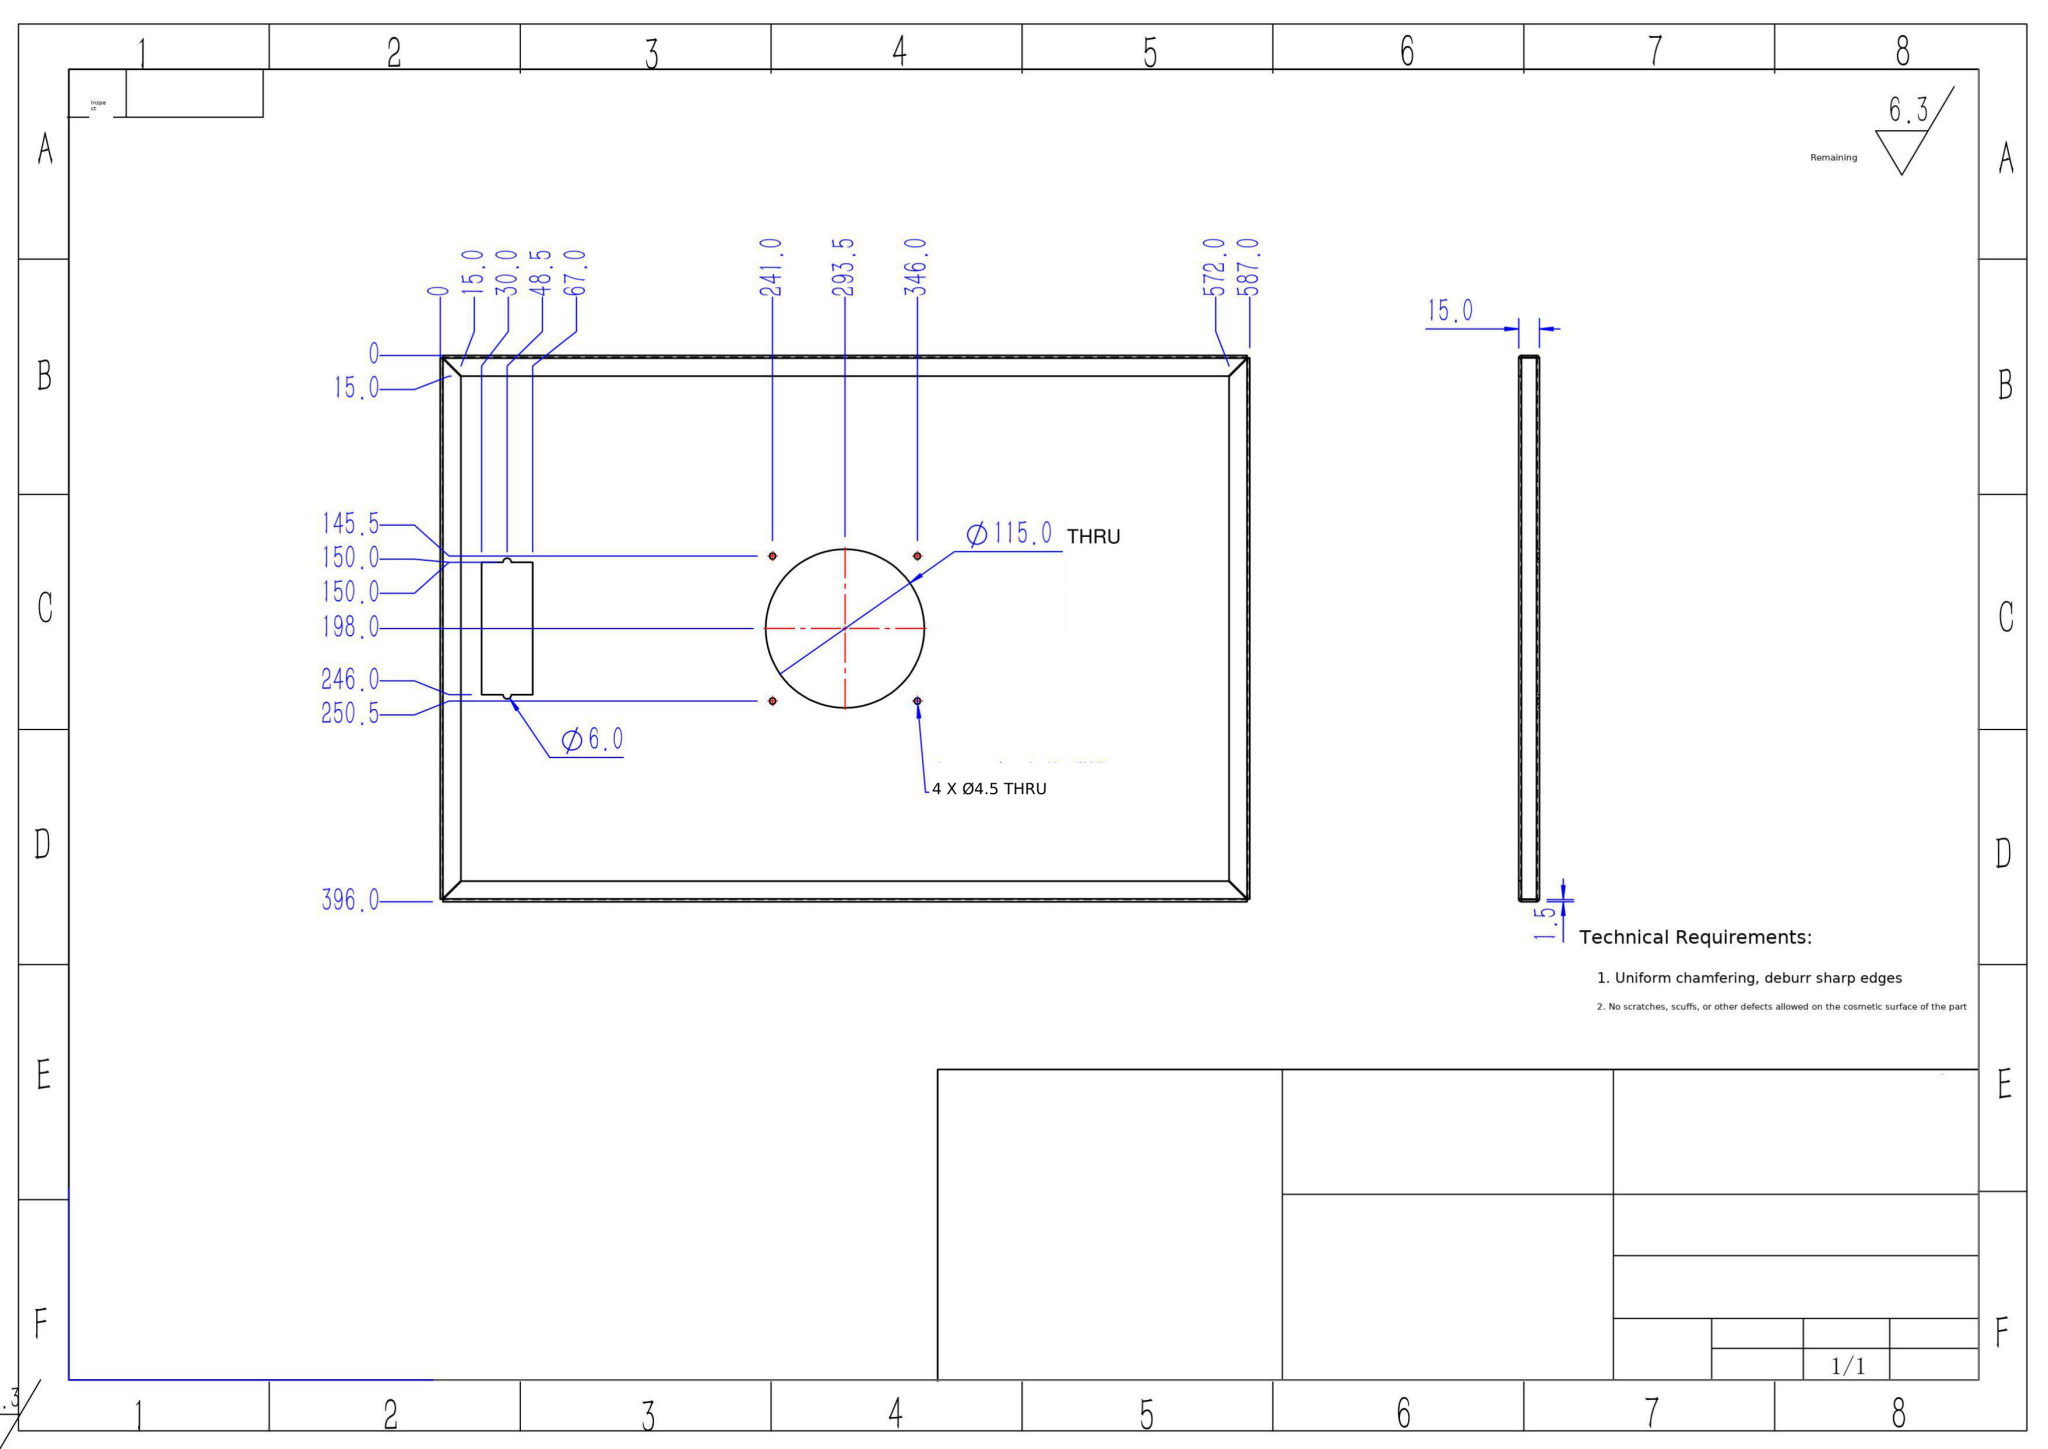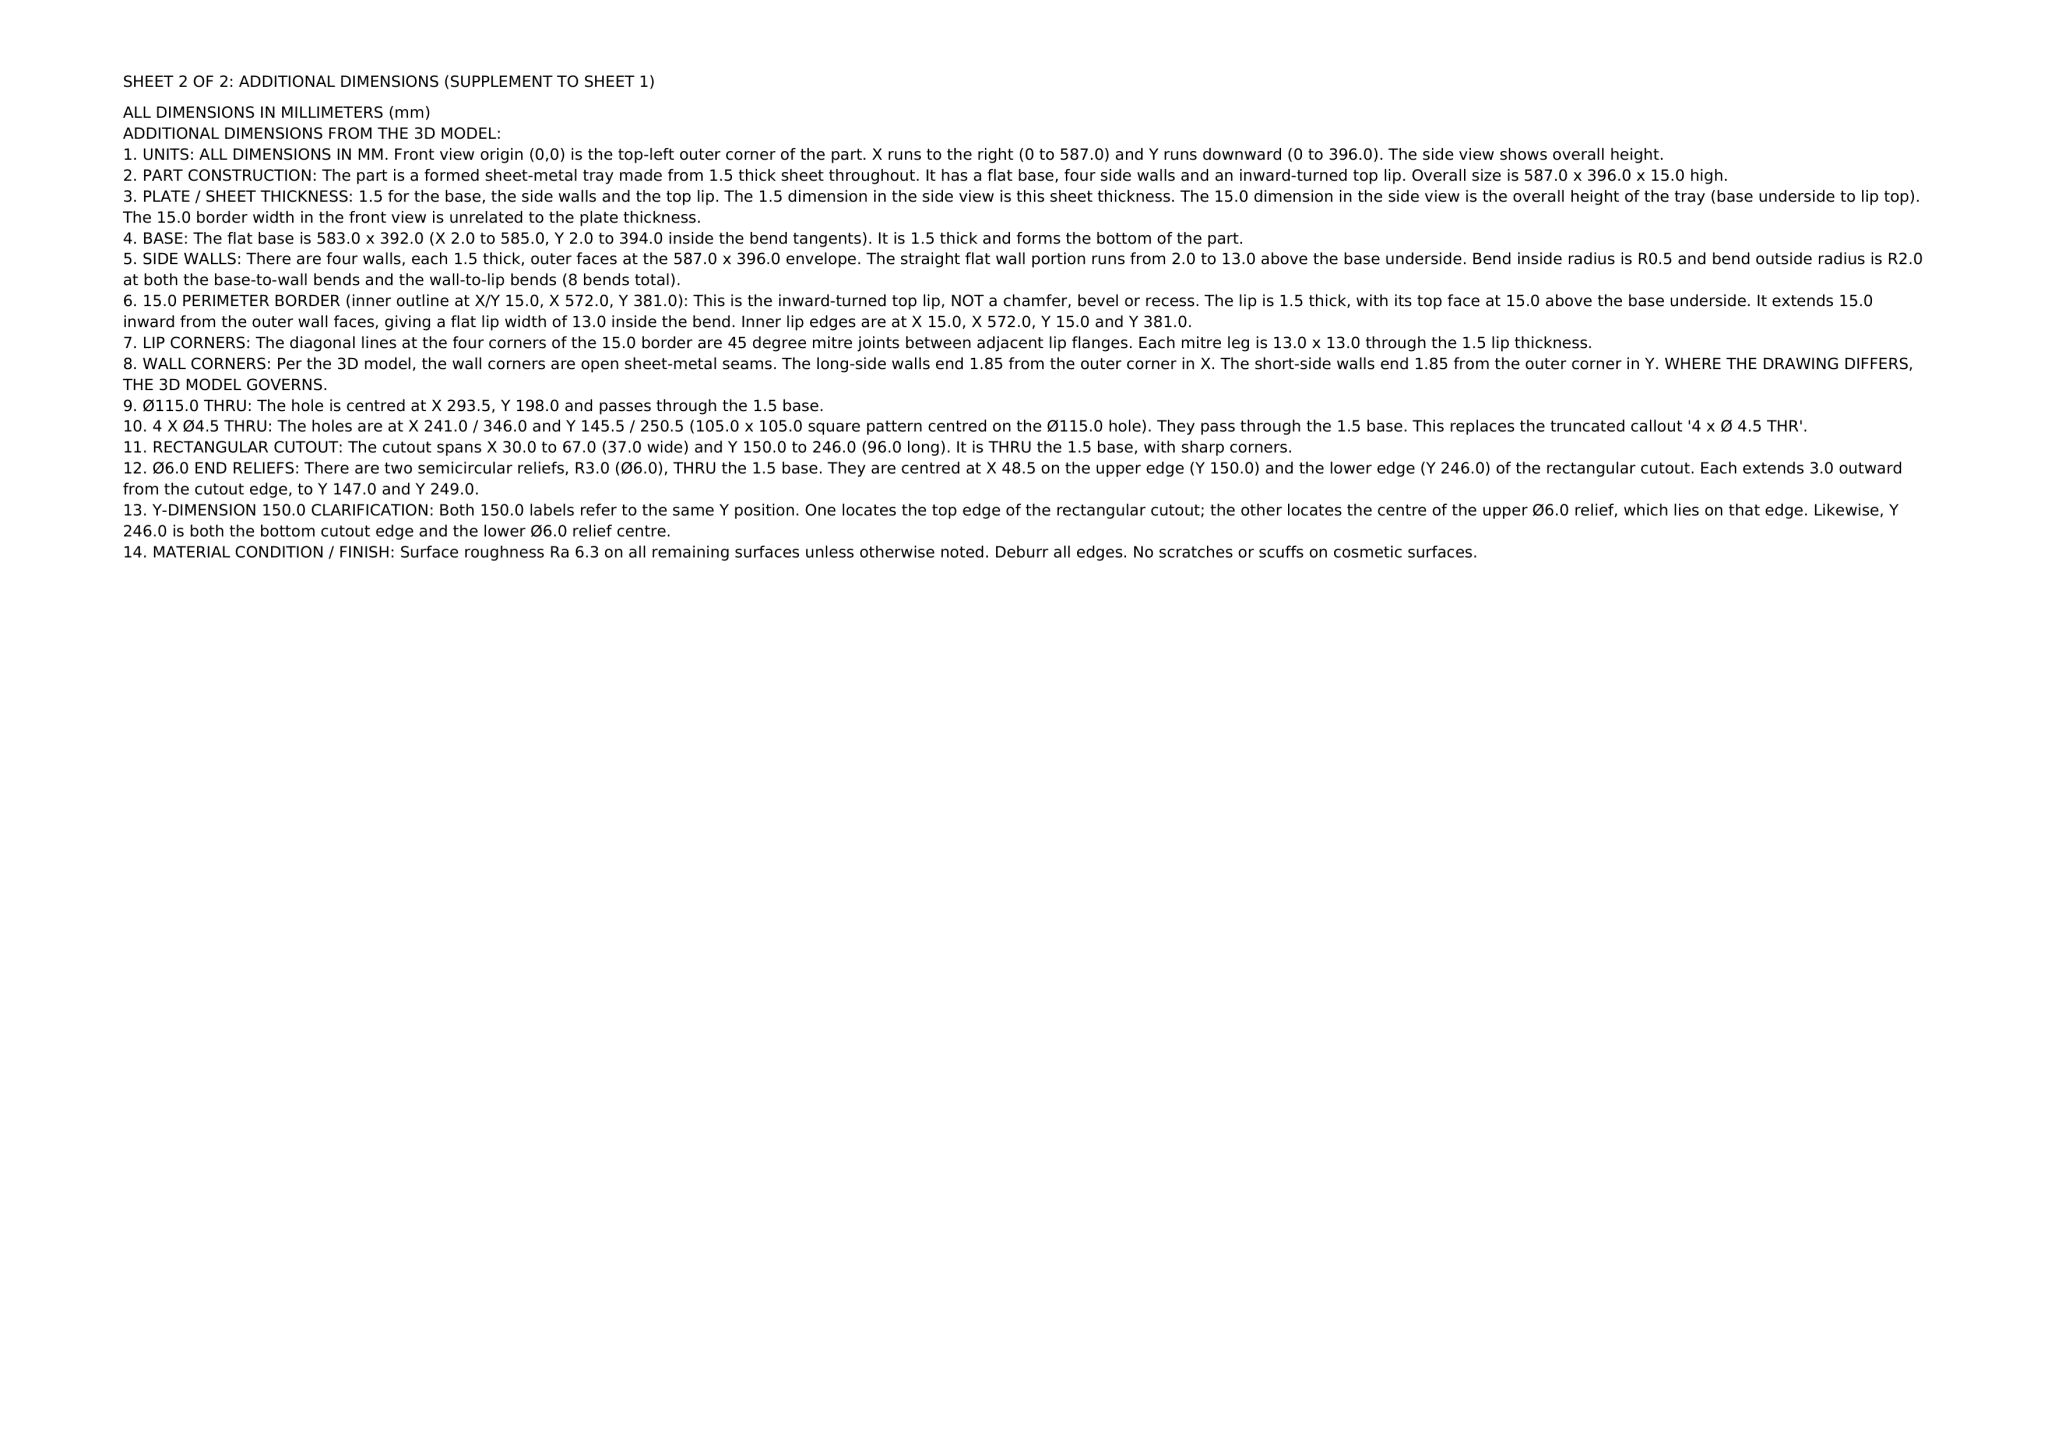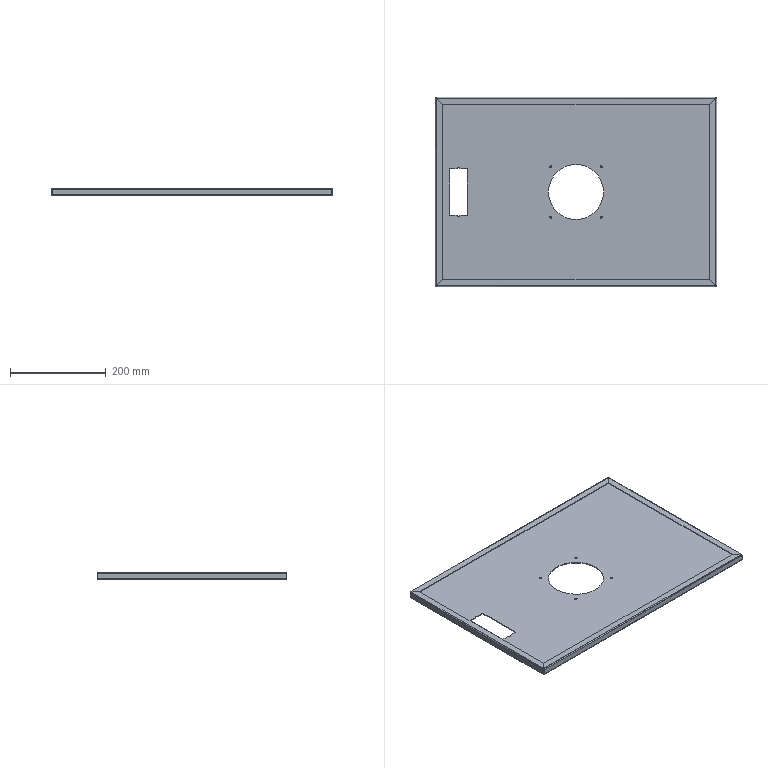Part | NX | mm | Rectangular Dual-Aperture Cover Plate | 1 solid | 88 faces | box 587 x 396 x 15 mm | volume 402394 mm3 | plane 44 | cylinder 28 | spline 16 | commonest cylinder face diameters 4.5 x8 4 x8 1 x8 115 x2 6 x2